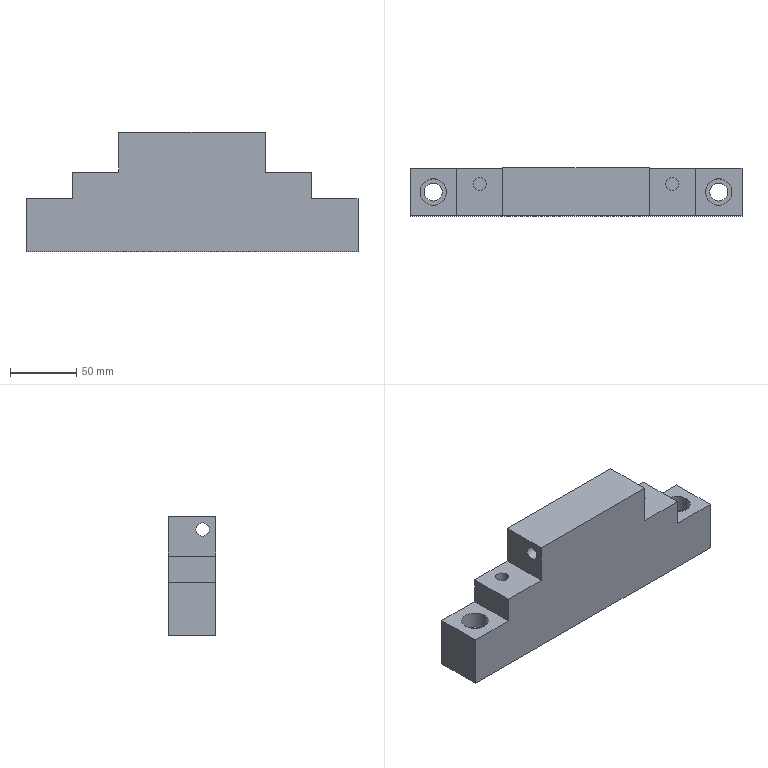Component | NX | SUPPORT | 1 solid | 25 faces | volume 581575 mm3 | plane 18 | cylinder 7 | commonest cylinder face diameters 10 x3 13.5 x2 20 x2